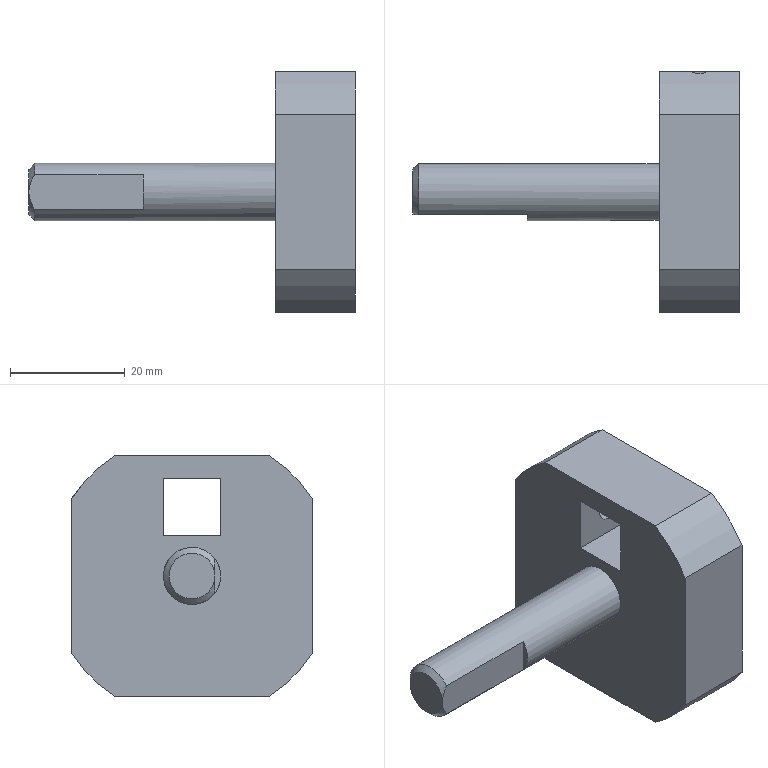Component | NX | 8_ROTATING_SHAFT | 1 solid | 20 faces | volume 25030 mm3 | plane 13 | cylinder 6 | cone 1 | commonest cylinder face diameters 50 x4 10 x1 4.2 x1